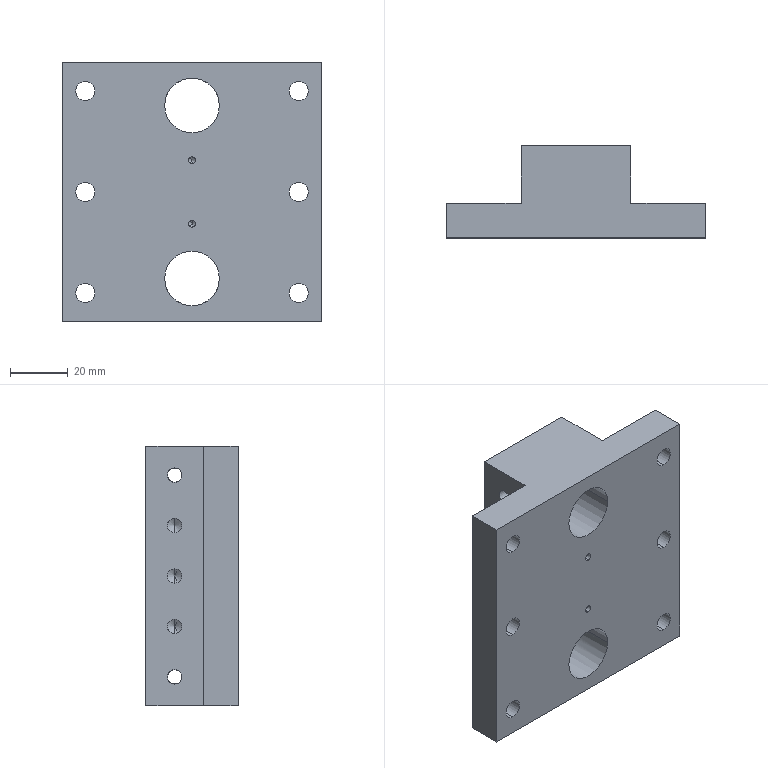Component | SolidWorks | QX1-12-V-BracketBase-1 | 1 solid | 102 faces | volume 141628 mm3 | cylinder 56 | cone 36 | plane 10 | commonest cylinder face diameters 5 x20 3.3 x16 6.6 x12 2.5 x4 19 x4 | material 6061 Alloy